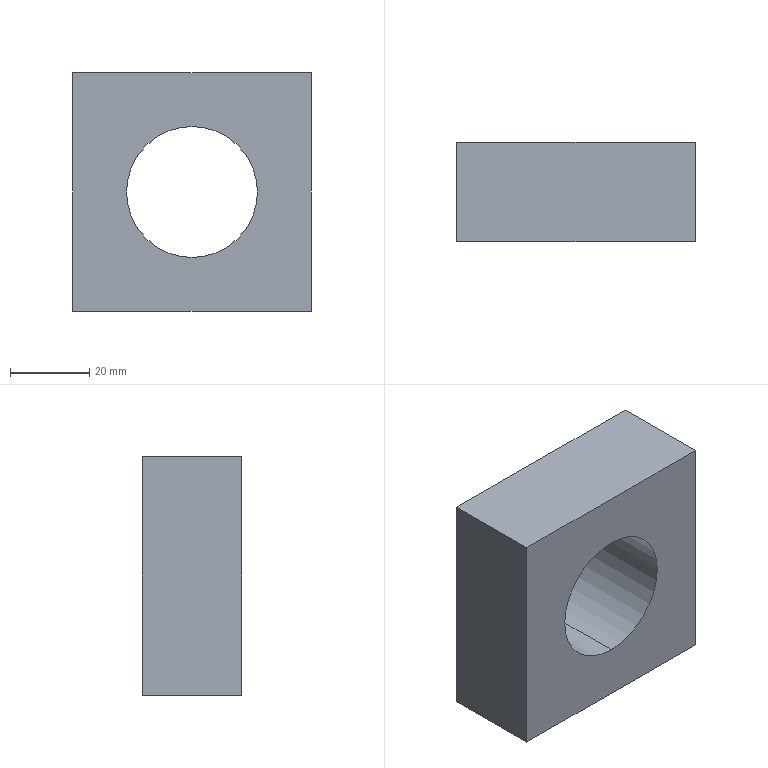Component | SolidWorks | JF21-80.1-1-3(_)-1-SOLID50-1 | 1 solid | 8 faces | box 60 x 25 x 60 mm | volume 68618 mm3 | plane 6 | cylinder 2 | commonest cylinder face diameters 33 x2
STEP:
#1=COLOUR_RGB('',0.7922,0.8196,0.9333);
#2=FILL_AREA_STYLE_COLOUR('',#1);
#3=FILL_AREA_STYLE('',(#2));
#4=SURFACE_STYLE_FILL_AREA(#3);
#5=SURFACE_SIDE_STYLE('',(#4));
#6=SURFACE_STYLE_USAGE(.BOTH.,#5);
#7=PRESENTATION_STYLE_ASSIGNMENT((#6));
#8=CARTESIAN_POINT('',(0.,-63.189,9.39));
#9=VERTEX_POINT('',#8);
#10=CARTESIAN_POINT('',(0.,-63.189,10.689));
#11=VERTEX_POINT('',#10);
#12=CARTESIAN_POINT('',(0.,-63.189,10.039));
#13=DIRECTION('',(0.,1.,0.));
#14=DIRECTION('',(0.,0.,1.));
#15=AXIS2_PLACEMENT_3D('',#12,#13,#14);
#16=CIRCLE('',#15,0.6496);
#17=EDGE_CURVE('',#9,#11,#16,.T.);
#18=ORIENTED_EDGE('',*,*,#17,.F.);
#19=CARTESIAN_POINT('',(0.,-62.205,9.39));
#20=VERTEX_POINT('',#19);
#21=CARTESIAN_POINT('',(0.,-62.205,9.39));
#22=DIRECTION('',(0.,1.,0.));
#23=VECTOR('',#22,39.37);
#24=LINE('',#21,#23);
#25=EDGE_CURVE('',#9,#20,#24,.T.);
#26=ORIENTED_EDGE('',*,*,#25,.T.);
#27=CARTESIAN_POINT('',(0.,-62.205,10.689));
#28=VERTEX_POINT('',#27);
#29=CARTESIAN_POINT('',(0.,-62.205,10.039));
#30=DIRECTION('',(0.,1.,0.));
#31=DIRECTION('',(0.,0.,1.));
#32=AXIS2_PLACEMENT_3D('',#29,#30,#31);
#33=CIRCLE('',#32,0.6496);
#34=EDGE_CURVE('',#20,#28,#33,.T.);
#35=ORIENTED_EDGE('',*,*,#34,.T.);
#36=CARTESIAN_POINT('',(0.,-62.205,10.689));
#37=DIRECTION('',(0.,1.,0.));
#38=VECTOR('',#37,39.37);
#39=LINE('',#36,#38);
#40=EDGE_CURVE('',#11,#28,#39,.T.);
#41=ORIENTED_EDGE('',*,*,#40,.F.);
#42=EDGE_LOOP('',(#18,#26,#35,#41));
#43=FACE_OUTER_BOUND('',#42,.T.);
#44=CARTESIAN_POINT('',(0.,-62.205,10.039));
#45=DIRECTION('',(0.,1.,0.));
#46=DIRECTION('',(0.,0.,-1.));
#47=AXIS2_PLACEMENT_3D('',#44,#45,#46);
#48=CYLINDRICAL_SURFACE('',#47,0.6496);
#49=ADVANCED_FACE('',(#43),#48,.F.);
#50=CARTESIAN_POINT('',(-1.181,-63.189,11.22));
#51=VERTEX_POINT('',#50);
#52=CARTESIAN_POINT('',(-1.181,-63.189,8.858));
#53=VERTEX_POINT('',#52);
#54=CARTESIAN_POINT('',(-1.181,-63.189,8.858));
#55=DIRECTION('',(0.,0.,-1.));
#56=VECTOR('',#55,39.37);
#57=LINE('',#54,#56);
#58=EDGE_CURVE('',#51,#53,#57,.T.);
#59=ORIENTED_EDGE('',*,*,#58,.F.);
#60=CARTESIAN_POINT('',(-1.181,-62.205,11.22));
#61=VERTEX_POINT('',#60);
#62=CARTESIAN_POINT('',(-1.181,-66.53,11.22));
#63=DIRECTION('',(0.,1.,0.));
#64=VECTOR('',#63,39.37);
#65=LINE('',#62,#64);
#66=EDGE_CURVE('',#51,#61,#65,.T.);
#67=ORIENTED_EDGE('',*,*,#66,.T.);
#68=CARTESIAN_POINT('',(-1.181,-62.205,8.858));
#69=VERTEX_POINT('',#68);
#70=CARTESIAN_POINT('',(-1.181,-62.205,8.858));
#71=DIRECTION('',(-0.,0.,1.));
#72=VECTOR('',#71,39.37);
#73=LINE('',#70,#72);
#74=EDGE_CURVE('',#69,#61,#73,.T.);
#75=ORIENTED_EDGE('',*,*,#74,.F.);
#76=CARTESIAN_POINT('',(-1.181,-66.53,8.858));
#77=DIRECTION('',(0.,1.,0.));
#78=VECTOR('',#77,39.37);
#79=LINE('',#76,#78);
#80=EDGE_CURVE('',#53,#69,#79,.T.);
#81=ORIENTED_EDGE('',*,*,#80,.F.);
#82=EDGE_LOOP('',(#59,#67,#75,#81));
#83=FACE_OUTER_BOUND('',#82,.T.);
#84=CARTESIAN_POINT('',(-1.181,-66.53,8.858));
#85=DIRECTION('',(-1.,0.,-0.));
#86=DIRECTION('',(0.,0.,-1.));
#87=AXIS2_PLACEMENT_3D('',#84,#85,#86);
#88=PLANE('',#87);
#89=ADVANCED_FACE('',(#83),#88,.T.);
#90=CARTESIAN_POINT('',(1.181,-63.189,8.858));
#91=VERTEX_POINT('',#90);
#92=CARTESIAN_POINT('',(-1.181,-63.189,8.858));
#93=DIRECTION('',(1.,0.,0.));
#94=VECTOR('',#93,39.37);
#95=LINE('',#92,#94);
#96=EDGE_CURVE('',#53,#91,#95,.T.);
#97=ORIENTED_EDGE('',*,*,#96,.F.);
#98=ORIENTED_EDGE('',*,*,#80,.T.);
#99=CARTESIAN_POINT('',(1.181,-62.205,8.858));
#100=VERTEX_POINT('',#99);
#101=CARTESIAN_POINT('',(-1.181,-62.205,8.858));
#102=DIRECTION('',(-1.,0.,0.));
#103=VECTOR('',#102,39.37);
#104=LINE('',#101,#103);
#105=EDGE_CURVE('',#100,#69,#104,.T.);
#106=ORIENTED_EDGE('',*,*,#105,.F.);
#107=CARTESIAN_POINT('',(1.181,-66.53,8.858));
#108=DIRECTION('',(0.,1.,0.));
#109=VECTOR('',#108,39.37);
#110=LINE('',#107,#109);
#111=EDGE_CURVE('',#91,#100,#110,.T.);
#112=ORIENTED_EDGE('',*,*,#111,.F.);
#113=EDGE_LOOP('',(#97,#98,#106,#112));
#114=FACE_OUTER_BOUND('',#113,.T.);
#115=CARTESIAN_POINT('',(-1.181,-66.53,8.858));
#116=DIRECTION('',(0.,0.,-1.));
#117=DIRECTION('',(1.,0.,0.));
#118=AXIS2_PLACEMENT_3D('',#115,#116,#117);
#119=PLANE('',#118);
#120=ADVANCED_FACE('',(#114),#119,.T.);
#121=CARTESIAN_POINT('',(1.181,-63.189,11.22));
#122=VERTEX_POINT('',#121);
#123=CARTESIAN_POINT('',(1.181,-63.189,8.858));
#124=DIRECTION('',(0.,0.,1.));
#125=VECTOR('',#124,39.37);
#126=LINE('',#123,#125);
#127=EDGE_CURVE('',#91,#122,#126,.T.);
#128=ORIENTED_EDGE('',*,*,#127,.F.);
#129=ORIENTED_EDGE('',*,*,#111,.T.);
#130=CARTESIAN_POINT('',(1.181,-62.205,11.22));
#131=VERTEX_POINT('',#130);
#132=CARTESIAN_POINT('',(1.181,-62.205,8.858));
#133=DIRECTION('',(-0.,0.,-1.));
#134=VECTOR('',#133,39.37);
#135=LINE('',#132,#134);
#136=EDGE_CURVE('',#131,#100,#135,.T.);
#137=ORIENTED_EDGE('',*,*,#136,.F.);
#138=CARTESIAN_POINT('',(1.181,-66.53,11.22));
#139=DIRECTION('',(0.,1.,0.));
#140=VECTOR('',#139,39.37);
#141=LINE('',#138,#140);
#142=EDGE_CURVE('',#122,#131,#141,.T.);
#143=ORIENTED_EDGE('',*,*,#142,.F.);
#144=EDGE_LOOP('',(#128,#129,#137,#143));
#145=FACE_OUTER_BOUND('',#144,.T.);
#146=CARTESIAN_POINT('',(1.181,-66.53,8.858));
#147=DIRECTION('',(1.,0.,-0.));
#148=DIRECTION('',(0.,0.,1.));
#149=AXIS2_PLACEMENT_3D('',#146,#147,#148);
#150=PLANE('',#149);
#151=ADVANCED_FACE('',(#145),#150,.T.);
#152=CARTESIAN_POINT('',(-1.181,-63.189,11.22));
#153=DIRECTION('',(-1.,0.,0.));
#154=VECTOR('',#153,39.37);
#155=LINE('',#152,#154);
#156=EDGE_CURVE('',#122,#51,#155,.T.);
#157=ORIENTED_EDGE('',*,*,#156,.F.);
#158=ORIENTED_EDGE('',*,*,#142,.T.);
#159=CARTESIAN_POINT('',(-1.181,-62.205,11.22));
#160=DIRECTION('',(1.,0.,0.));
#161=VECTOR('',#160,39.37);
#162=LINE('',#159,#161);
#163=EDGE_CURVE('',#61,#131,#162,.T.);
#164=ORIENTED_EDGE('',*,*,#163,.F.);
#165=ORIENTED_EDGE('',*,*,#66,.F.);
#166=EDGE_LOOP('',(#157,#158,#164,#165));
#167=FACE_OUTER_BOUND('',#166,.T.);
#168=CARTESIAN_POINT('',(-1.181,-66.53,11.22));
#169=DIRECTION('',(0.,0.,1.));
#170=DIRECTION('',(-1.,0.,0.));
#171=AXIS2_PLACEMENT_3D('',#168,#169,#170);
#172=PLANE('',#171);
#173=ADVANCED_FACE('',(#167),#172,.T.);
#174=CARTESIAN_POINT('',(0.,-62.205,10.039));
#175=DIRECTION('',(0.,1.,0.));
#176=DIRECTION('',(0.,0.,1.));
#177=AXIS2_PLACEMENT_3D('',#174,#175,#176);
#178=CIRCLE('',#177,0.6496);
#179=EDGE_CURVE('',#28,#20,#178,.T.);
#180=ORIENTED_EDGE('',*,*,#179,.F.);
#181=ORIENTED_EDGE('',*,*,#34,.F.);
#182=EDGE_LOOP('',(#180,#181));
#183=FACE_BOUND('',#182,.T.);
#184=ORIENTED_EDGE('',*,*,#74,.T.);
#185=ORIENTED_EDGE('',*,*,#163,.T.);
#186=ORIENTED_EDGE('',*,*,#136,.T.);
#187=ORIENTED_EDGE('',*,*,#105,.T.);
#188=EDGE_LOOP('',(#184,#185,#186,#187));
#189=FACE_OUTER_BOUND('',#188,.T.);
#190=CARTESIAN_POINT('',(-1.181,-62.205,11.22));
#191=DIRECTION('',(0.,1.,0.));
#192=DIRECTION('',(0.,0.,-1.));
#193=AXIS2_PLACEMENT_3D('',#190,#191,#192);
#194=PLANE('',#193);
#195=ADVANCED_FACE('',(#183,#189),#194,.T.);
#196=CARTESIAN_POINT('',(0.,-63.189,10.039));
#197=DIRECTION('',(0.,1.,0.));
#198=DIRECTION('',(0.,0.,1.));
#199=AXIS2_PLACEMENT_3D('',#196,#197,#198);
#200=CIRCLE('',#199,0.6496);
#201=EDGE_CURVE('',#11,#9,#200,.T.);
#202=ORIENTED_EDGE('',*,*,#201,.T.);
#203=ORIENTED_EDGE('',*,*,#17,.T.);
#204=EDGE_LOOP('',(#202,#203));
#205=FACE_BOUND('',#204,.T.);
#206=ORIENTED_EDGE('',*,*,#58,.T.);
#207=ORIENTED_EDGE('',*,*,#96,.T.);
#208=ORIENTED_EDGE('',*,*,#127,.T.);
#209=ORIENTED_EDGE('',*,*,#156,.T.);
#210=EDGE_LOOP('',(#206,#207,#208,#209));
#211=FACE_OUTER_BOUND('',#210,.T.);
#212=CARTESIAN_POINT('',(-12.598,-63.189,21.654));
#213=DIRECTION('',(0.,1.,0.));
#214=DIRECTION('',(0.,0.,-1.));
#215=AXIS2_PLACEMENT_3D('',#212,#213,#214);
#216=PLANE('',#215);
#217=ADVANCED_FACE('',(#205,#211),#216,.F.);
#218=ORIENTED_EDGE('',*,*,#25,.F.);
#219=ORIENTED_EDGE('',*,*,#201,.F.);
#220=ORIENTED_EDGE('',*,*,#40,.T.);
#221=ORIENTED_EDGE('',*,*,#179,.T.);
#222=EDGE_LOOP('',(#218,#219,#220,#221));
#223=FACE_OUTER_BOUND('',#222,.T.);
#224=CARTESIAN_POINT('',(0.,-62.205,10.039));
#225=DIRECTION('',(0.,1.,0.));
#226=DIRECTION('',(0.,0.,-1.));
#227=AXIS2_PLACEMENT_3D('',#224,#225,#226);
#228=CYLINDRICAL_SURFACE('',#227,0.6496);
#229=ADVANCED_FACE('',(#223),#228,.F.);
#230=CLOSED_SHELL('',(#49,#89,#120,#151,#173,#195,#217,#229));
#231=MANIFOLD_SOLID_BREP('',#230);
#232=STYLED_ITEM('',(#7),#231);
#233=(LENGTH_UNIT()NAMED_UNIT(*)SI_UNIT($,.METRE.));
#234=LENGTH_MEASURE_WITH_UNIT(LENGTH_MEASURE(0.0254),#233);
#235=DIMENSIONAL_EXPONENTS(1.,0.,0.,0.,0.,0.,0.);
#236=(CONVERSION_BASED_UNIT('',#234)LENGTH_UNIT()NAMED_UNIT(#235));
#237=UNCERTAINTY_MEASURE_WITH_UNIT(LENGTH_MEASURE(0.00001),#236,'','');
#238=(NAMED_UNIT(*)PLANE_ANGLE_UNIT()SI_UNIT($,.RADIAN.));
#239=(NAMED_UNIT(*)SI_UNIT($,.STERADIAN.)SOLID_ANGLE_UNIT());
#240=(GEOMETRIC_REPRESENTATION_CONTEXT(3)GLOBAL_UNCERTAINTY_ASSIGNED_CONTEXT((#237))GLOBAL_UNIT_ASSIGNED_CONTEXT((#236,#238,#239))REPRESENTATION_CONTEXT('',''));
#241=MECHANICAL_DESIGN_GEOMETRIC_PRESENTATION_REPRESENTATION('',(#232),#240);
#242=CARTESIAN_POINT('',(0.,0.,0.));
#243=DIRECTION('',(0.,0.,1.));
#244=DIRECTION('',(1.,0.,0.));
#245=AXIS2_PLACEMENT_3D('',#242,#243,#244);
#246=(LENGTH_UNIT()NAMED_UNIT(*)SI_UNIT($,.METRE.));
#247=LENGTH_MEASURE_WITH_UNIT(LENGTH_MEASURE(0.0254),#246);
#248=DIMENSIONAL_EXPONENTS(1.,0.,0.,0.,0.,0.,0.);
#249=(CONVERSION_BASED_UNIT('',#247)LENGTH_UNIT()NAMED_UNIT(#248));
#250=UNCERTAINTY_MEASURE_WITH_UNIT(LENGTH_MEASURE(0.00001),#249,'','');
#251=(NAMED_UNIT(*)PLANE_ANGLE_UNIT()SI_UNIT($,.RADIAN.));
#252=(NAMED_UNIT(*)SI_UNIT($,.STERADIAN.)SOLID_ANGLE_UNIT());
#253=(GEOMETRIC_REPRESENTATION_CONTEXT(3)GLOBAL_UNCERTAINTY_ASSIGNED_CONTEXT((#250))GLOBAL_UNIT_ASSIGNED_CONTEXT((#249,#251,#252))REPRESENTATION_CONTEXT('',''));
#254=ADVANCED_BREP_SHAPE_REPRESENTATION('',(#231,#245),#253);
#255=PRESENTATION_LAYER_ASSIGNMENT('','',(#232));